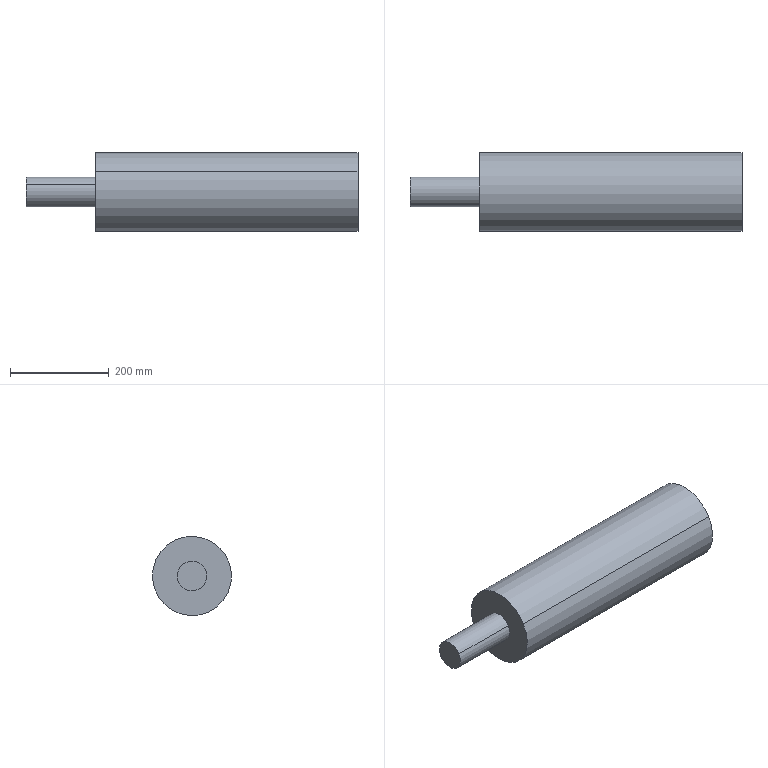Component | SolidWorks | DriveShaft-1 | 1 solid | 10 faces | box 671.23 x 160 x 160 mm | volume 9585327 mm3 | cylinder 6 | plane 4 | commonest cylinder face diameters 60 x4 160 x2
build123d program:
from build123d import *

# Parameters (mm, degrees)
SKETCH1_R                       = 31
REPAIR_REMOVEINNERJOURNAL_DEPTH = 57.056
SKETCH2_R                       = 30
REPAIR_SPINDLEBORE60_DEPTH      = 260.056


with BuildPart() as part:
    # Sketch1_2 → Revolve1 (revolve)
    with BuildSketch(Plane.XZ, mode=Mode.PRIVATE) as revolve1_sk:
        Polygon((30, 784.007), (0, 784.007), (0, 0), (30, 0), (30, 112.78), (80, 112.78), (80, 642.78), (30, 642.78), align=None)
    revolve(revolve1_sk.sketch.rotate(Axis((0, 0, 784.007), (0, 0, -1)), 180), axis=Axis((0, 0, 784.007), (0, 0, -1)))

    # Sketch1 → Repair_RemoveInnerJournal (cut, symmetric)
    with BuildSketch(Plane.XY.offset(55.724)):
        Circle(SKETCH1_R)
    extrude(amount=REPAIR_REMOVEINNERJOURNAL_DEPTH, both=True, mode=Mode.SUBTRACT)

    # Sketch2 → Repair_SpindleBore60 (cut, symmetric)
    with BuildSketch(Plane.XY.offset(372.724)):
        with Locations(Location((0, 0, 0), (0, 0, 180))):
            Circle(SKETCH2_R)
    extrude(amount=REPAIR_SPINDLEBORE60_DEPTH, both=True, mode=Mode.SUBTRACT)


solid = part.part

# Placed as in the assembly
solid = solid.moved(Location((-119.332, 1335.766, 1014.597), (0, -90, 0)))
STEP:
#1=COLOUR_RGB('',0.7922,0.8196,0.9333);
#2=FILL_AREA_STYLE_COLOUR('',#1);
#3=FILL_AREA_STYLE('',(#2));
#4=SURFACE_STYLE_FILL_AREA(#3);
#5=SURFACE_SIDE_STYLE('',(#4));
#6=SURFACE_STYLE_USAGE(.BOTH.,#5);
#7=PRESENTATION_STYLE_ASSIGNMENT((#6));
#8=CARTESIAN_POINT('',(-9.138,53.602,39.336));
#9=VERTEX_POINT('',#8);
#10=CARTESIAN_POINT('',(-9.138,51.577,40.553));
#11=VERTEX_POINT('',#10);
#12=CARTESIAN_POINT('',(-9.138,52.589,39.945));
#13=DIRECTION('',(1.,0.,0.));
#14=DIRECTION('',(0.,-0.8572,0.515));
#15=AXIS2_PLACEMENT_3D('',#12,#13,#14);
#16=CIRCLE('',#15,1.181);
#17=EDGE_CURVE('',#9,#11,#16,.T.);
#18=ORIENTED_EDGE('',*,*,#17,.T.);
#19=CARTESIAN_POINT('',(-29.611,51.577,40.553));
#20=VERTEX_POINT('',#19);
#21=CARTESIAN_POINT('',(-9.134,51.577,40.553));
#22=DIRECTION('',(-1.,0.,0.));
#23=VECTOR('',#22,39.37);
#24=LINE('',#21,#23);
#25=EDGE_CURVE('',#11,#20,#24,.T.);
#26=ORIENTED_EDGE('',*,*,#25,.T.);
#27=CARTESIAN_POINT('',(-29.611,53.602,39.336));
#28=VERTEX_POINT('',#27);
#29=CARTESIAN_POINT('',(-29.611,52.589,39.945));
#30=DIRECTION('',(-1.,0.,0.));
#31=DIRECTION('',(0.,0.8572,-0.515));
#32=AXIS2_PLACEMENT_3D('',#29,#30,#31);
#33=CIRCLE('',#32,1.181);
#34=EDGE_CURVE('',#20,#28,#33,.T.);
#35=ORIENTED_EDGE('',*,*,#34,.T.);
#36=CARTESIAN_POINT('',(-9.134,53.602,39.336));
#37=DIRECTION('',(-1.,0.,0.));
#38=VECTOR('',#37,39.37);
#39=LINE('',#36,#38);
#40=EDGE_CURVE('',#9,#28,#39,.T.);
#41=ORIENTED_EDGE('',*,*,#40,.F.);
#42=EDGE_LOOP('',(#18,#26,#35,#41));
#43=FACE_OUTER_BOUND('',#42,.T.);
#44=CARTESIAN_POINT('',(-9.134,52.589,39.945));
#45=DIRECTION('',(-1.,0.,0.));
#46=DIRECTION('',(0.,0.8572,-0.515));
#47=AXIS2_PLACEMENT_3D('',#44,#45,#46);
#48=CYLINDRICAL_SURFACE('',#47,1.181);
#49=ADVANCED_FACE('',(#43),#48,.F.);
#50=CARTESIAN_POINT('',(-30.004,49.889,41.567));
#51=VERTEX_POINT('',#50);
#52=CARTESIAN_POINT('',(-30.004,55.289,38.323));
#53=VERTEX_POINT('',#52);
#54=CARTESIAN_POINT('',(-30.004,52.589,39.945));
#55=DIRECTION('',(1.,0.,0.));
#56=DIRECTION('',(0.,-0.8572,0.515));
#57=AXIS2_PLACEMENT_3D('',#54,#55,#56);
#58=CIRCLE('',#57,3.15);
#59=EDGE_CURVE('',#51,#53,#58,.T.);
#60=ORIENTED_EDGE('',*,*,#59,.T.);
#61=CARTESIAN_POINT('',(-9.138,55.289,38.323));
#62=VERTEX_POINT('',#61);
#63=CARTESIAN_POINT('',(-35.565,55.289,38.323));
#64=DIRECTION('',(1.,0.,0.));
#65=VECTOR('',#64,39.37);
#66=LINE('',#63,#65);
#67=EDGE_CURVE('',#53,#62,#66,.T.);
#68=ORIENTED_EDGE('',*,*,#67,.T.);
#69=CARTESIAN_POINT('',(-9.138,49.889,41.567));
#70=VERTEX_POINT('',#69);
#71=CARTESIAN_POINT('',(-9.138,52.589,39.945));
#72=DIRECTION('',(1.,0.,0.));
#73=DIRECTION('',(0.,-0.8572,0.515));
#74=AXIS2_PLACEMENT_3D('',#71,#72,#73);
#75=CIRCLE('',#74,3.15);
#76=EDGE_CURVE('',#70,#62,#75,.T.);
#77=ORIENTED_EDGE('',*,*,#76,.F.);
#78=CARTESIAN_POINT('',(-35.565,49.889,41.567));
#79=DIRECTION('',(1.,0.,0.));
#80=VECTOR('',#79,39.37);
#81=LINE('',#78,#80);
#82=EDGE_CURVE('',#51,#70,#81,.T.);
#83=ORIENTED_EDGE('',*,*,#82,.F.);
#84=EDGE_LOOP('',(#60,#68,#77,#83));
#85=FACE_OUTER_BOUND('',#84,.T.);
#86=CARTESIAN_POINT('',(-35.565,52.589,39.945));
#87=DIRECTION('',(1.,0.,0.));
#88=DIRECTION('',(0.,-0.8572,0.515));
#89=AXIS2_PLACEMENT_3D('',#86,#87,#88);
#90=CYLINDRICAL_SURFACE('',#89,3.15);
#91=ADVANCED_FACE('',(#85),#90,.T.);
#92=CARTESIAN_POINT('',(-35.565,51.577,40.553));
#93=VERTEX_POINT('',#92);
#94=CARTESIAN_POINT('',(-35.565,53.602,39.336));
#95=VERTEX_POINT('',#94);
#96=CARTESIAN_POINT('',(-35.565,52.589,39.945));
#97=DIRECTION('',(1.,0.,0.));
#98=DIRECTION('',(0.,-0.8572,0.515));
#99=AXIS2_PLACEMENT_3D('',#96,#97,#98);
#100=CIRCLE('',#99,1.181);
#101=EDGE_CURVE('',#93,#95,#100,.T.);
#102=ORIENTED_EDGE('',*,*,#101,.T.);
#103=CARTESIAN_POINT('',(-30.004,53.602,39.336));
#104=VERTEX_POINT('',#103);
#105=CARTESIAN_POINT('',(-35.565,53.602,39.336));
#106=DIRECTION('',(1.,0.,0.));
#107=VECTOR('',#106,39.37);
#108=LINE('',#105,#107);
#109=EDGE_CURVE('',#95,#104,#108,.T.);
#110=ORIENTED_EDGE('',*,*,#109,.T.);
#111=CARTESIAN_POINT('',(-30.004,51.577,40.553));
#112=VERTEX_POINT('',#111);
#113=CARTESIAN_POINT('',(-30.004,52.589,39.945));
#114=DIRECTION('',(1.,0.,0.));
#115=DIRECTION('',(0.,-0.8572,0.515));
#116=AXIS2_PLACEMENT_3D('',#113,#114,#115);
#117=CIRCLE('',#116,1.181);
#118=EDGE_CURVE('',#112,#104,#117,.T.);
#119=ORIENTED_EDGE('',*,*,#118,.F.);
#120=CARTESIAN_POINT('',(-35.565,51.577,40.553));
#121=DIRECTION('',(1.,0.,0.));
#122=VECTOR('',#121,39.37);
#123=LINE('',#120,#122);
#124=EDGE_CURVE('',#93,#112,#123,.T.);
#125=ORIENTED_EDGE('',*,*,#124,.F.);
#126=EDGE_LOOP('',(#102,#110,#119,#125));
#127=FACE_OUTER_BOUND('',#126,.T.);
#128=CARTESIAN_POINT('',(-35.565,52.589,39.945));
#129=DIRECTION('',(1.,0.,0.));
#130=DIRECTION('',(0.,-0.8572,0.515));
#131=AXIS2_PLACEMENT_3D('',#128,#129,#130);
#132=CYLINDRICAL_SURFACE('',#131,1.181);
#133=ADVANCED_FACE('',(#127),#132,.T.);
#134=ORIENTED_EDGE('',*,*,#109,.F.);
#135=CARTESIAN_POINT('',(-35.565,52.589,39.945));
#136=DIRECTION('',(1.,0.,0.));
#137=DIRECTION('',(0.,-0.8572,0.515));
#138=AXIS2_PLACEMENT_3D('',#135,#136,#137);
#139=CIRCLE('',#138,1.181);
#140=EDGE_CURVE('',#95,#93,#139,.T.);
#141=ORIENTED_EDGE('',*,*,#140,.T.);
#142=ORIENTED_EDGE('',*,*,#124,.T.);
#143=CARTESIAN_POINT('',(-30.004,52.589,39.945));
#144=DIRECTION('',(1.,0.,0.));
#145=DIRECTION('',(0.,-0.8572,0.515));
#146=AXIS2_PLACEMENT_3D('',#143,#144,#145);
#147=CIRCLE('',#146,1.181);
#148=EDGE_CURVE('',#104,#112,#147,.T.);
#149=ORIENTED_EDGE('',*,*,#148,.F.);
#150=EDGE_LOOP('',(#134,#141,#142,#149));
#151=FACE_OUTER_BOUND('',#150,.T.);
#152=CARTESIAN_POINT('',(-35.565,52.589,39.945));
#153=DIRECTION('',(1.,0.,0.));
#154=DIRECTION('',(0.,-0.8572,0.515));
#155=AXIS2_PLACEMENT_3D('',#152,#153,#154);
#156=CYLINDRICAL_SURFACE('',#155,1.181);
#157=ADVANCED_FACE('',(#151),#156,.T.);
#158=ORIENTED_EDGE('',*,*,#101,.F.);
#159=ORIENTED_EDGE('',*,*,#140,.F.);
#160=EDGE_LOOP('',(#158,#159));
#161=FACE_OUTER_BOUND('',#160,.T.);
#162=CARTESIAN_POINT('',(-35.565,53.602,39.336));
#163=DIRECTION('',(-1.,0.,0.));
#164=DIRECTION('',(0.,0.8572,-0.515));
#165=AXIS2_PLACEMENT_3D('',#162,#163,#164);
#166=PLANE('',#165);
#167=ADVANCED_FACE('',(#161),#166,.T.);
#168=ORIENTED_EDGE('',*,*,#17,.F.);
#169=CARTESIAN_POINT('',(-9.138,52.589,39.945));
#170=DIRECTION('',(1.,0.,0.));
#171=DIRECTION('',(0.,-0.8572,0.515));
#172=AXIS2_PLACEMENT_3D('',#169,#170,#171);
#173=CIRCLE('',#172,1.181);
#174=EDGE_CURVE('',#11,#9,#173,.T.);
#175=ORIENTED_EDGE('',*,*,#174,.F.);
#176=EDGE_LOOP('',(#168,#175));
#177=FACE_BOUND('',#176,.T.);
#178=ORIENTED_EDGE('',*,*,#76,.T.);
#179=CARTESIAN_POINT('',(-9.138,52.589,39.945));
#180=DIRECTION('',(1.,0.,0.));
#181=DIRECTION('',(0.,-0.8572,0.515));
#182=AXIS2_PLACEMENT_3D('',#179,#180,#181);
#183=CIRCLE('',#182,3.15);
#184=EDGE_CURVE('',#62,#70,#183,.T.);
#185=ORIENTED_EDGE('',*,*,#184,.T.);
#186=EDGE_LOOP('',(#178,#185));
#187=FACE_OUTER_BOUND('',#186,.T.);
#188=CARTESIAN_POINT('',(-9.138,53.602,39.336));
#189=DIRECTION('',(1.,0.,0.));
#190=DIRECTION('',(0.,-0.8572,0.515));
#191=AXIS2_PLACEMENT_3D('',#188,#189,#190);
#192=PLANE('',#191);
#193=ADVANCED_FACE('',(#177,#187),#192,.T.);
#194=ORIENTED_EDGE('',*,*,#67,.F.);
#195=CARTESIAN_POINT('',(-30.004,52.589,39.945));
#196=DIRECTION('',(1.,0.,0.));
#197=DIRECTION('',(0.,-0.8572,0.515));
#198=AXIS2_PLACEMENT_3D('',#195,#196,#197);
#199=CIRCLE('',#198,3.15);
#200=EDGE_CURVE('',#53,#51,#199,.T.);
#201=ORIENTED_EDGE('',*,*,#200,.T.);
#202=ORIENTED_EDGE('',*,*,#82,.T.);
#203=ORIENTED_EDGE('',*,*,#184,.F.);
#204=EDGE_LOOP('',(#194,#201,#202,#203));
#205=FACE_OUTER_BOUND('',#204,.T.);
#206=CARTESIAN_POINT('',(-35.565,52.589,39.945));
#207=DIRECTION('',(1.,0.,0.));
#208=DIRECTION('',(0.,-0.8572,0.515));
#209=AXIS2_PLACEMENT_3D('',#206,#207,#208);
#210=CYLINDRICAL_SURFACE('',#209,3.15);
#211=ADVANCED_FACE('',(#205),#210,.T.);
#212=ORIENTED_EDGE('',*,*,#118,.T.);
#213=ORIENTED_EDGE('',*,*,#148,.T.);
#214=EDGE_LOOP('',(#212,#213));
#215=FACE_BOUND('',#214,.T.);
#216=ORIENTED_EDGE('',*,*,#59,.F.);
#217=ORIENTED_EDGE('',*,*,#200,.F.);
#218=EDGE_LOOP('',(#216,#217));
#219=FACE_OUTER_BOUND('',#218,.T.);
#220=CARTESIAN_POINT('',(-30.004,55.289,38.323));
#221=DIRECTION('',(-1.,0.,0.));
#222=DIRECTION('',(0.,0.8572,-0.515));
#223=AXIS2_PLACEMENT_3D('',#220,#221,#222);
#224=PLANE('',#223);
#225=ADVANCED_FACE('',(#215,#219),#224,.T.);
#226=ORIENTED_EDGE('',*,*,#25,.F.);
#227=ORIENTED_EDGE('',*,*,#174,.T.);
#228=ORIENTED_EDGE('',*,*,#40,.T.);
#229=CARTESIAN_POINT('',(-29.611,52.589,39.945));
#230=DIRECTION('',(-1.,0.,0.));
#231=DIRECTION('',(0.,0.8572,-0.515));
#232=AXIS2_PLACEMENT_3D('',#229,#230,#231);
#233=CIRCLE('',#232,1.181);
#234=EDGE_CURVE('',#28,#20,#233,.T.);
#235=ORIENTED_EDGE('',*,*,#234,.T.);
#236=EDGE_LOOP('',(#226,#227,#228,#235));
#237=FACE_OUTER_BOUND('',#236,.T.);
#238=CARTESIAN_POINT('',(-9.134,52.589,39.945));
#239=DIRECTION('',(-1.,0.,0.));
#240=DIRECTION('',(0.,0.8572,-0.515));
#241=AXIS2_PLACEMENT_3D('',#238,#239,#240);
#242=CYLINDRICAL_SURFACE('',#241,1.181);
#243=ADVANCED_FACE('',(#237),#242,.F.);
#244=ORIENTED_EDGE('',*,*,#234,.F.);
#245=ORIENTED_EDGE('',*,*,#34,.F.);
#246=EDGE_LOOP('',(#244,#245));
#247=FACE_OUTER_BOUND('',#246,.T.);
#248=CARTESIAN_POINT('',(-29.611,52.589,39.945));
#249=DIRECTION('',(-1.,0.,0.));
#250=DIRECTION('',(0.,0.8572,-0.515));
#251=AXIS2_PLACEMENT_3D('',#248,#249,#250);
#252=PLANE('',#251);
#253=ADVANCED_FACE('',(#247),#252,.F.);
#254=CLOSED_SHELL('',(#49,#91,#133,#157,#167,#193,#211,#225,#243,#253));
#255=MANIFOLD_SOLID_BREP('',#254);
#256=STYLED_ITEM('',(#7),#255);
#257=(LENGTH_UNIT()NAMED_UNIT(*)SI_UNIT($,.METRE.));
#258=LENGTH_MEASURE_WITH_UNIT(LENGTH_MEASURE(0.0254),#257);
#259=DIMENSIONAL_EXPONENTS(1.,0.,0.,0.,0.,0.,0.);
#260=(CONVERSION_BASED_UNIT('',#258)LENGTH_UNIT()NAMED_UNIT(#259));
#261=UNCERTAINTY_MEASURE_WITH_UNIT(LENGTH_MEASURE(0.00001),#260,'','');
#262=(NAMED_UNIT(*)PLANE_ANGLE_UNIT()SI_UNIT($,.RADIAN.));
#263=(NAMED_UNIT(*)SI_UNIT($,.STERADIAN.)SOLID_ANGLE_UNIT());
#264=(GEOMETRIC_REPRESENTATION_CONTEXT(3)GLOBAL_UNCERTAINTY_ASSIGNED_CONTEXT((#261))GLOBAL_UNIT_ASSIGNED_CONTEXT((#260,#262,#263))REPRESENTATION_CONTEXT('',''));
#265=MECHANICAL_DESIGN_GEOMETRIC_PRESENTATION_REPRESENTATION('',(#256),#264);
#266=PRESENTATION_LAYER_ASSIGNMENT('','',(#256));
#267=CARTESIAN_POINT('',(0.,0.,0.));
#268=DIRECTION('',(0.,0.,1.));
#269=DIRECTION('',(1.,0.,0.));
#270=AXIS2_PLACEMENT_3D('',#267,#268,#269);
#271=(LENGTH_UNIT()NAMED_UNIT(*)SI_UNIT($,.METRE.));
#272=LENGTH_MEASURE_WITH_UNIT(LENGTH_MEASURE(0.0254),#271);
#273=DIMENSIONAL_EXPONENTS(1.,0.,0.,0.,0.,0.,0.);
#274=(CONVERSION_BASED_UNIT('',#272)LENGTH_UNIT()NAMED_UNIT(#273));
#275=UNCERTAINTY_MEASURE_WITH_UNIT(LENGTH_MEASURE(0.00001),#274,'','');
#276=(NAMED_UNIT(*)PLANE_ANGLE_UNIT()SI_UNIT($,.RADIAN.));
#277=(NAMED_UNIT(*)SI_UNIT($,.STERADIAN.)SOLID_ANGLE_UNIT());
#278=(GEOMETRIC_REPRESENTATION_CONTEXT(3)GLOBAL_UNCERTAINTY_ASSIGNED_CONTEXT((#275))GLOBAL_UNIT_ASSIGNED_CONTEXT((#274,#276,#277))REPRESENTATION_CONTEXT('',''));
#279=ADVANCED_BREP_SHAPE_REPRESENTATION('',(#255,#270),#278);